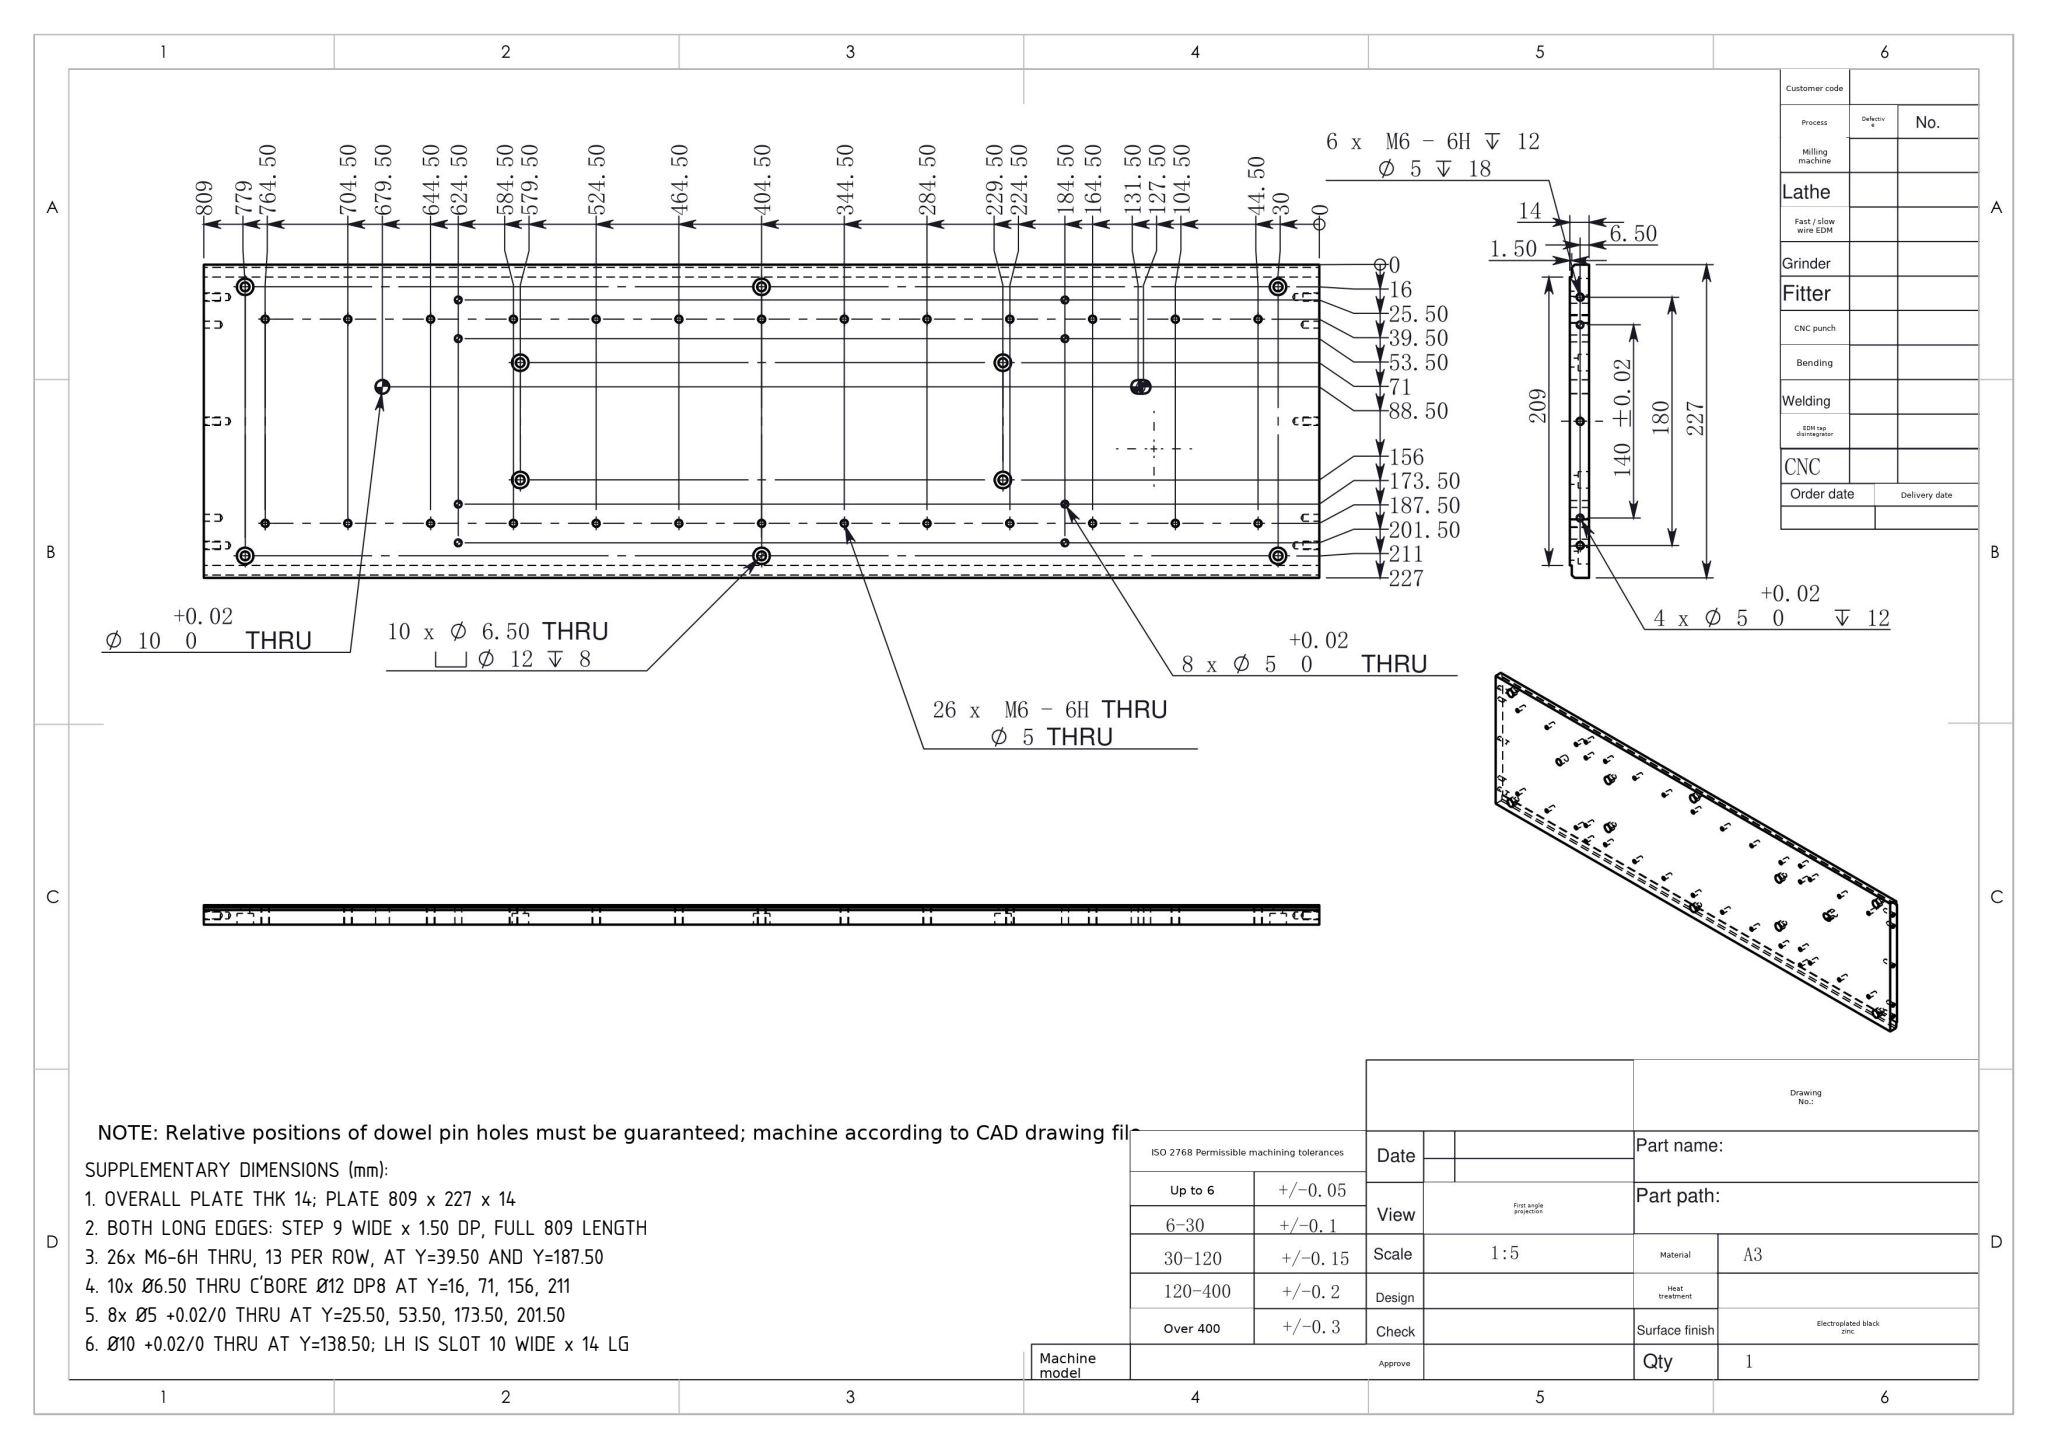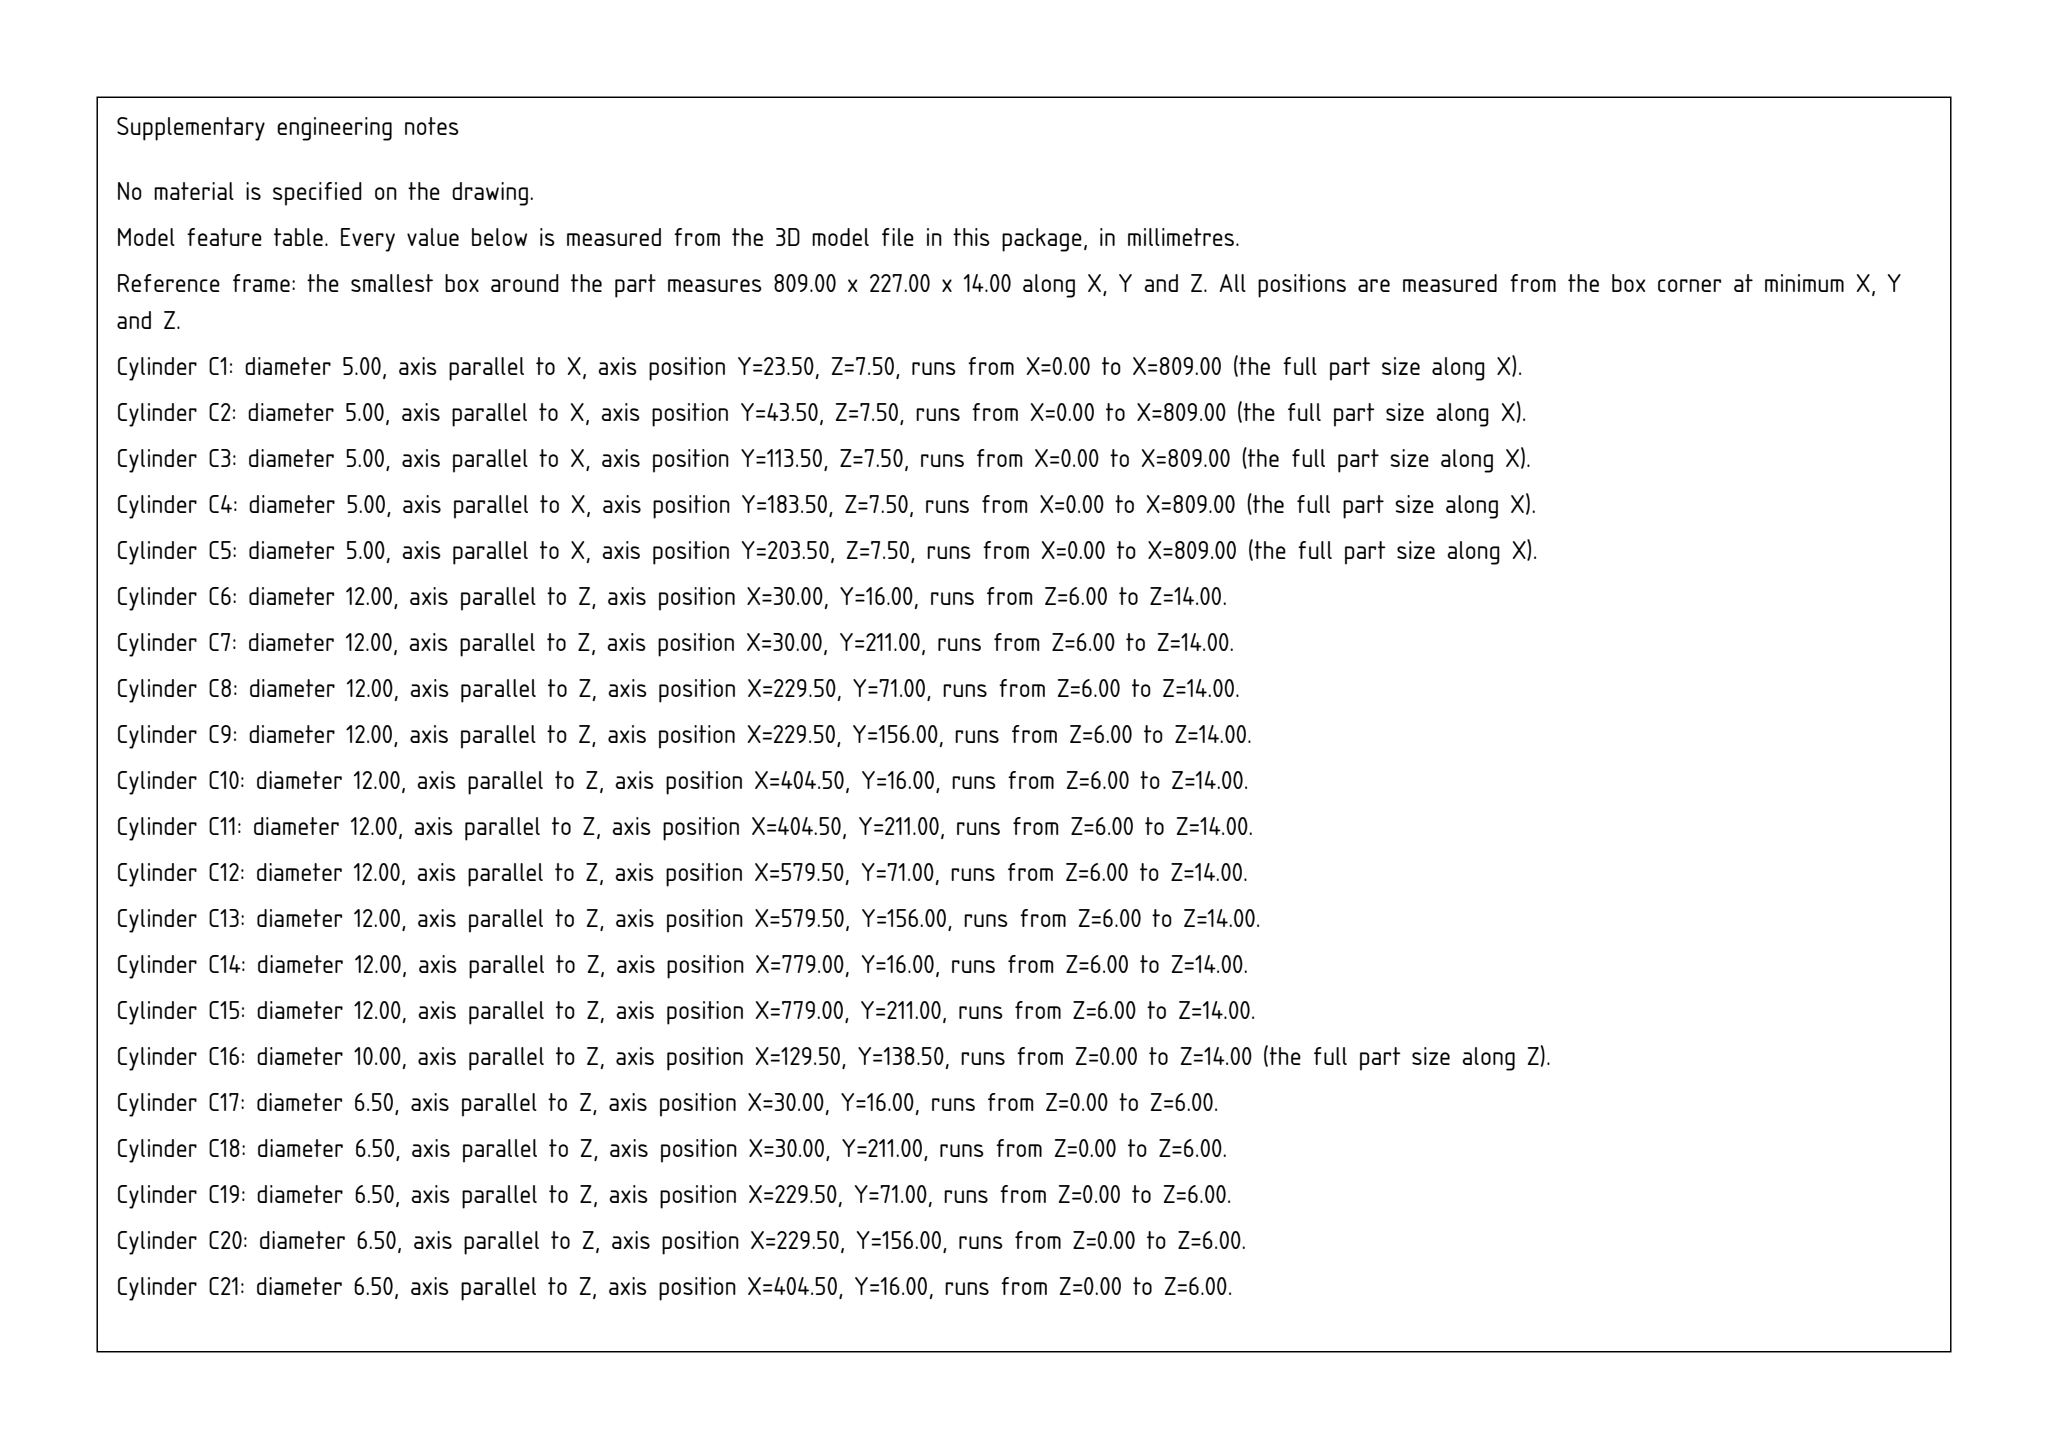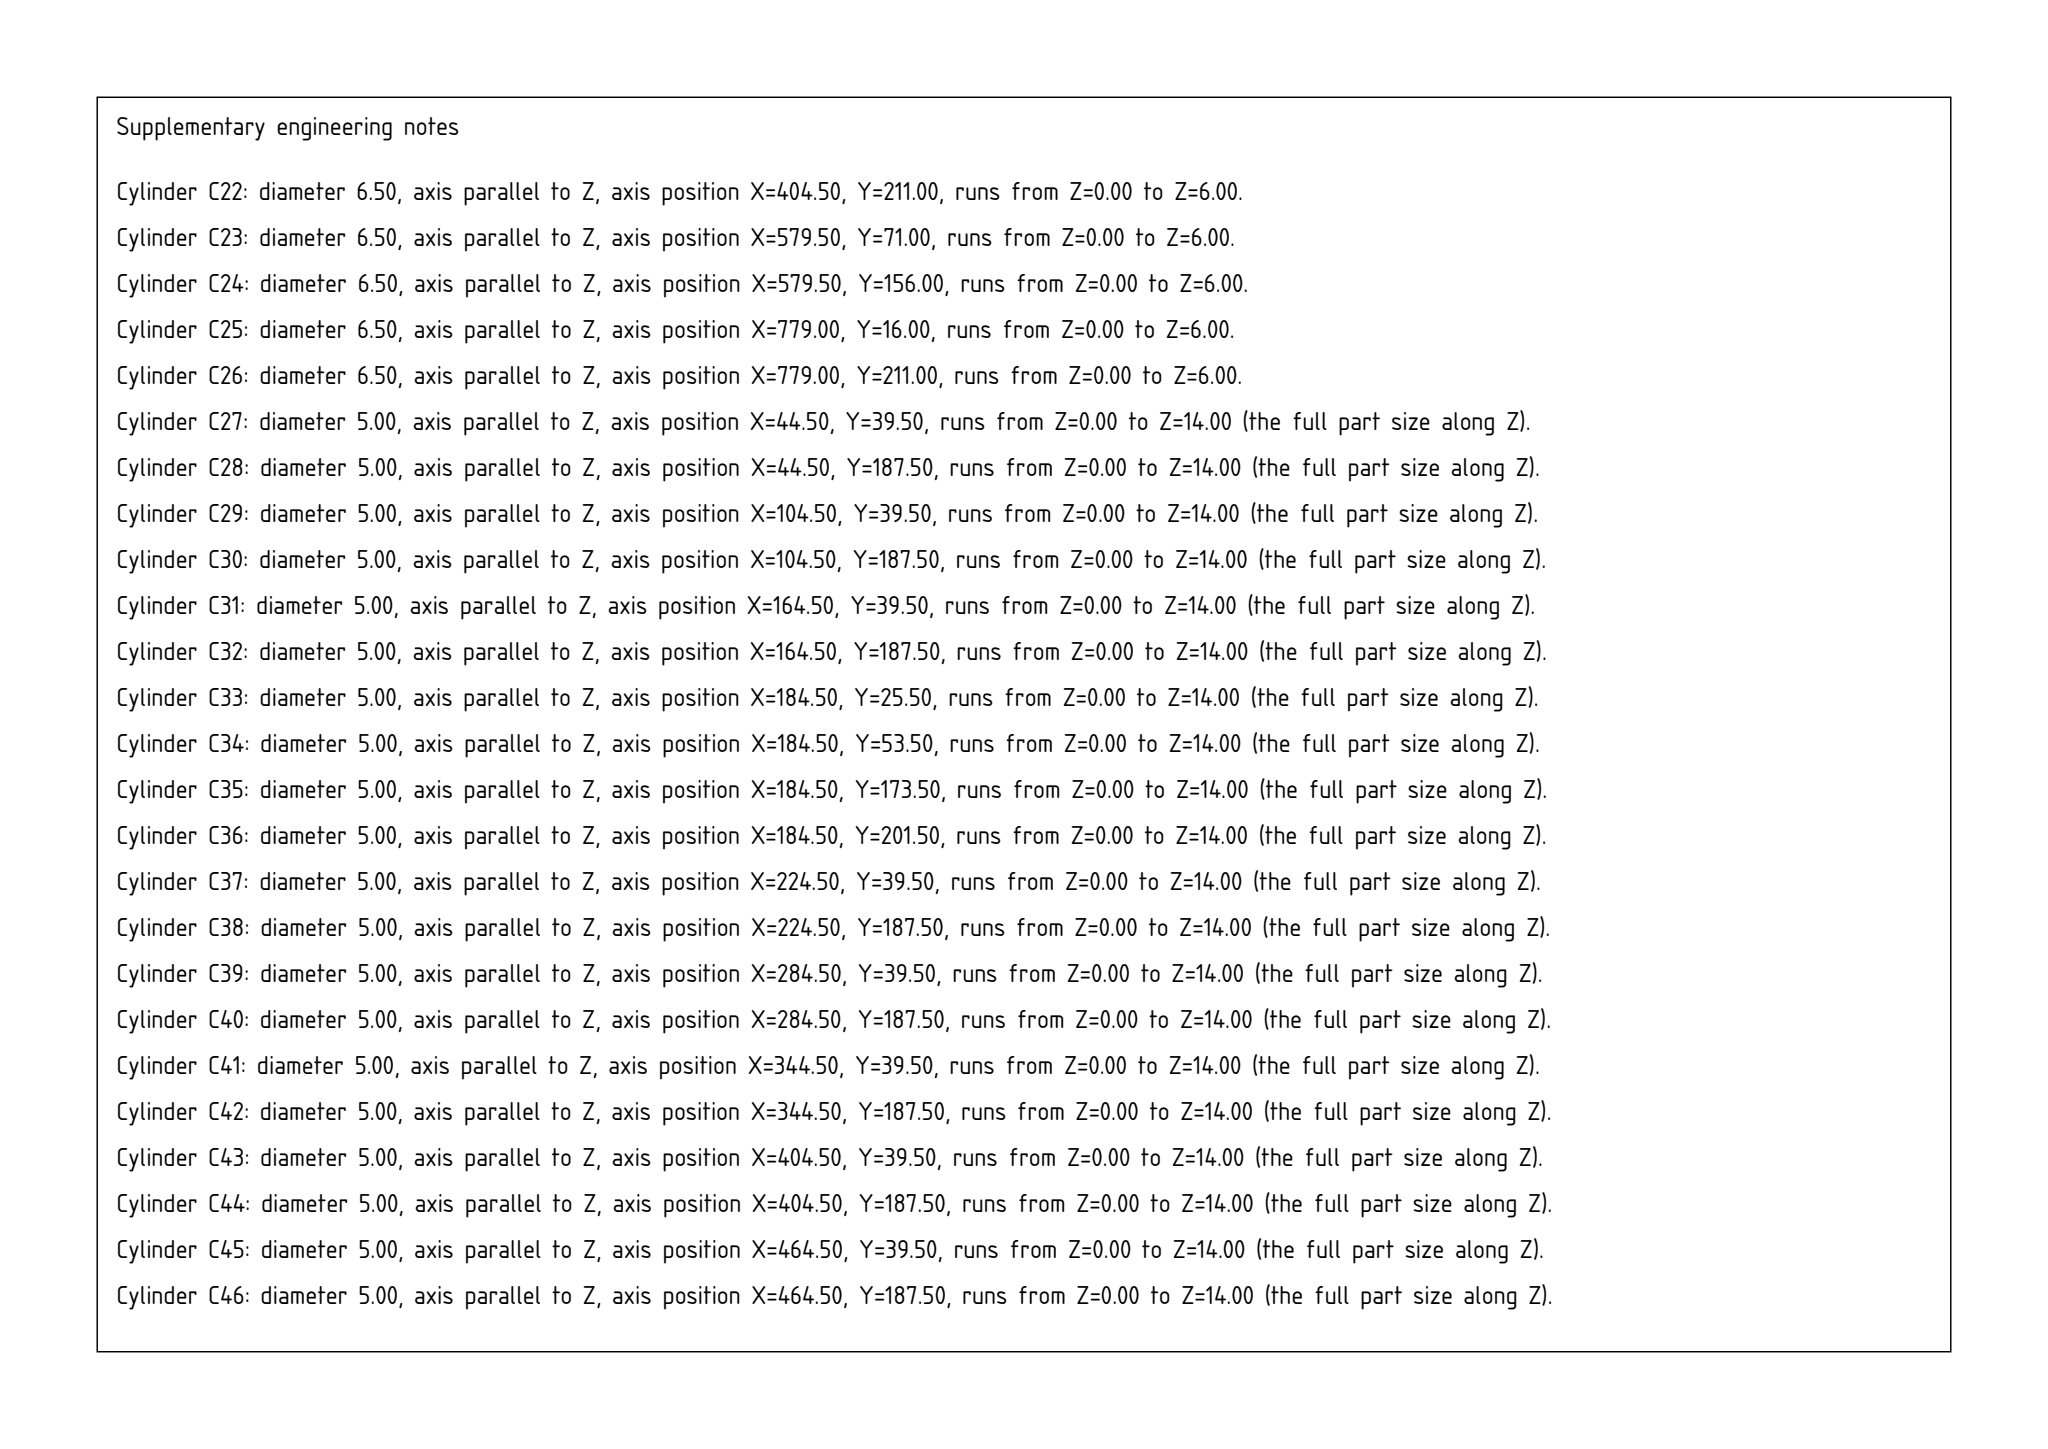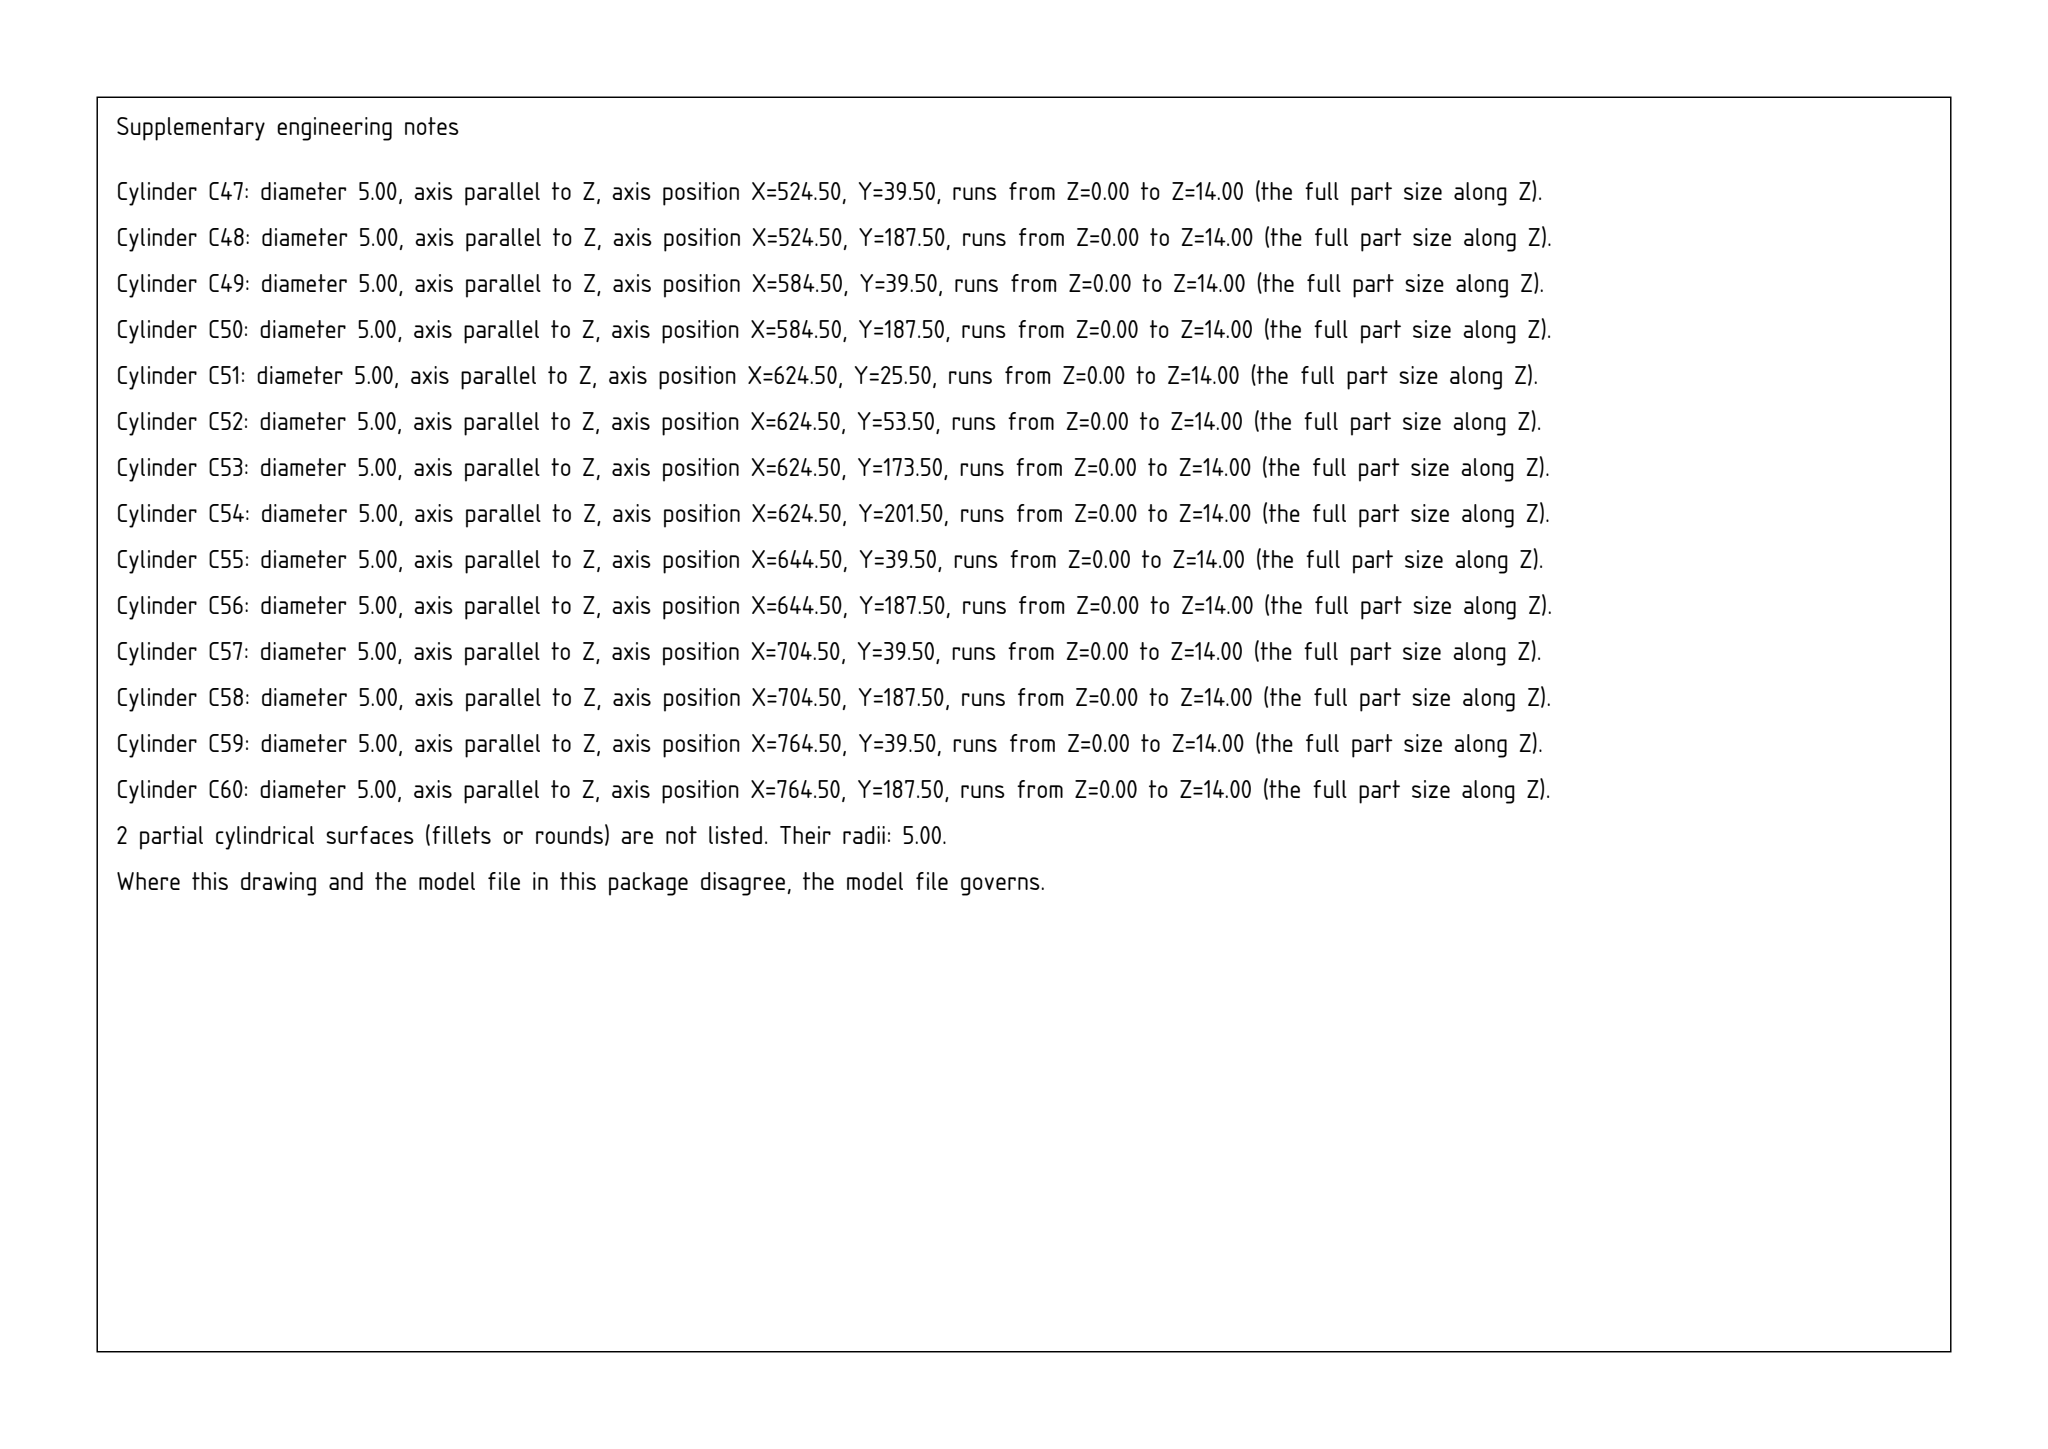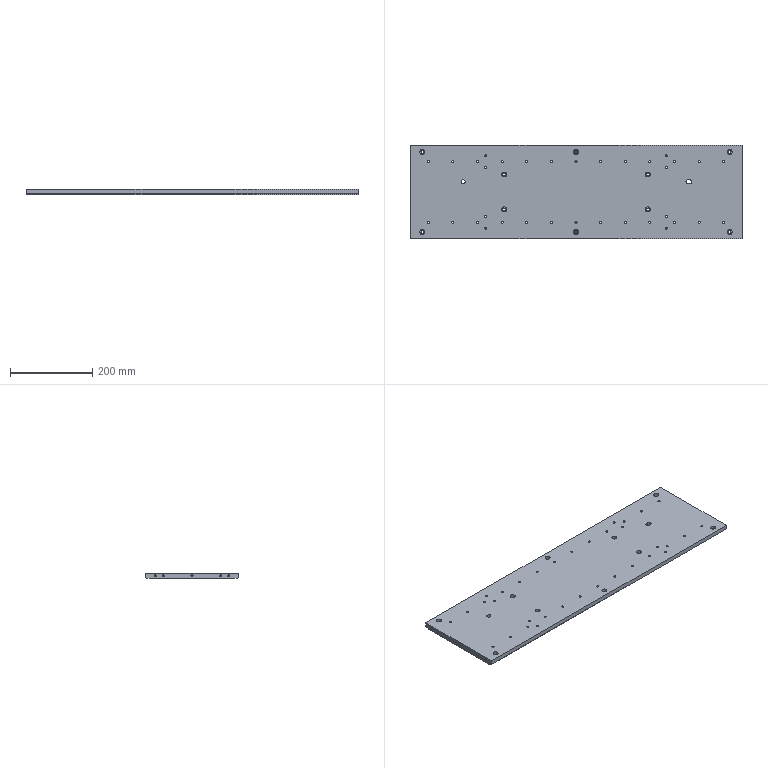Part | SolidWorks | mm | 1 solid | 177 faces | box 809 x 227 x 14 mm | volume 2519618 mm3 | cylinder 133 | plane 24 | cone 20 | commonest cylinder face diameters 5 x88 12 x20 6.5 x20 10 x5